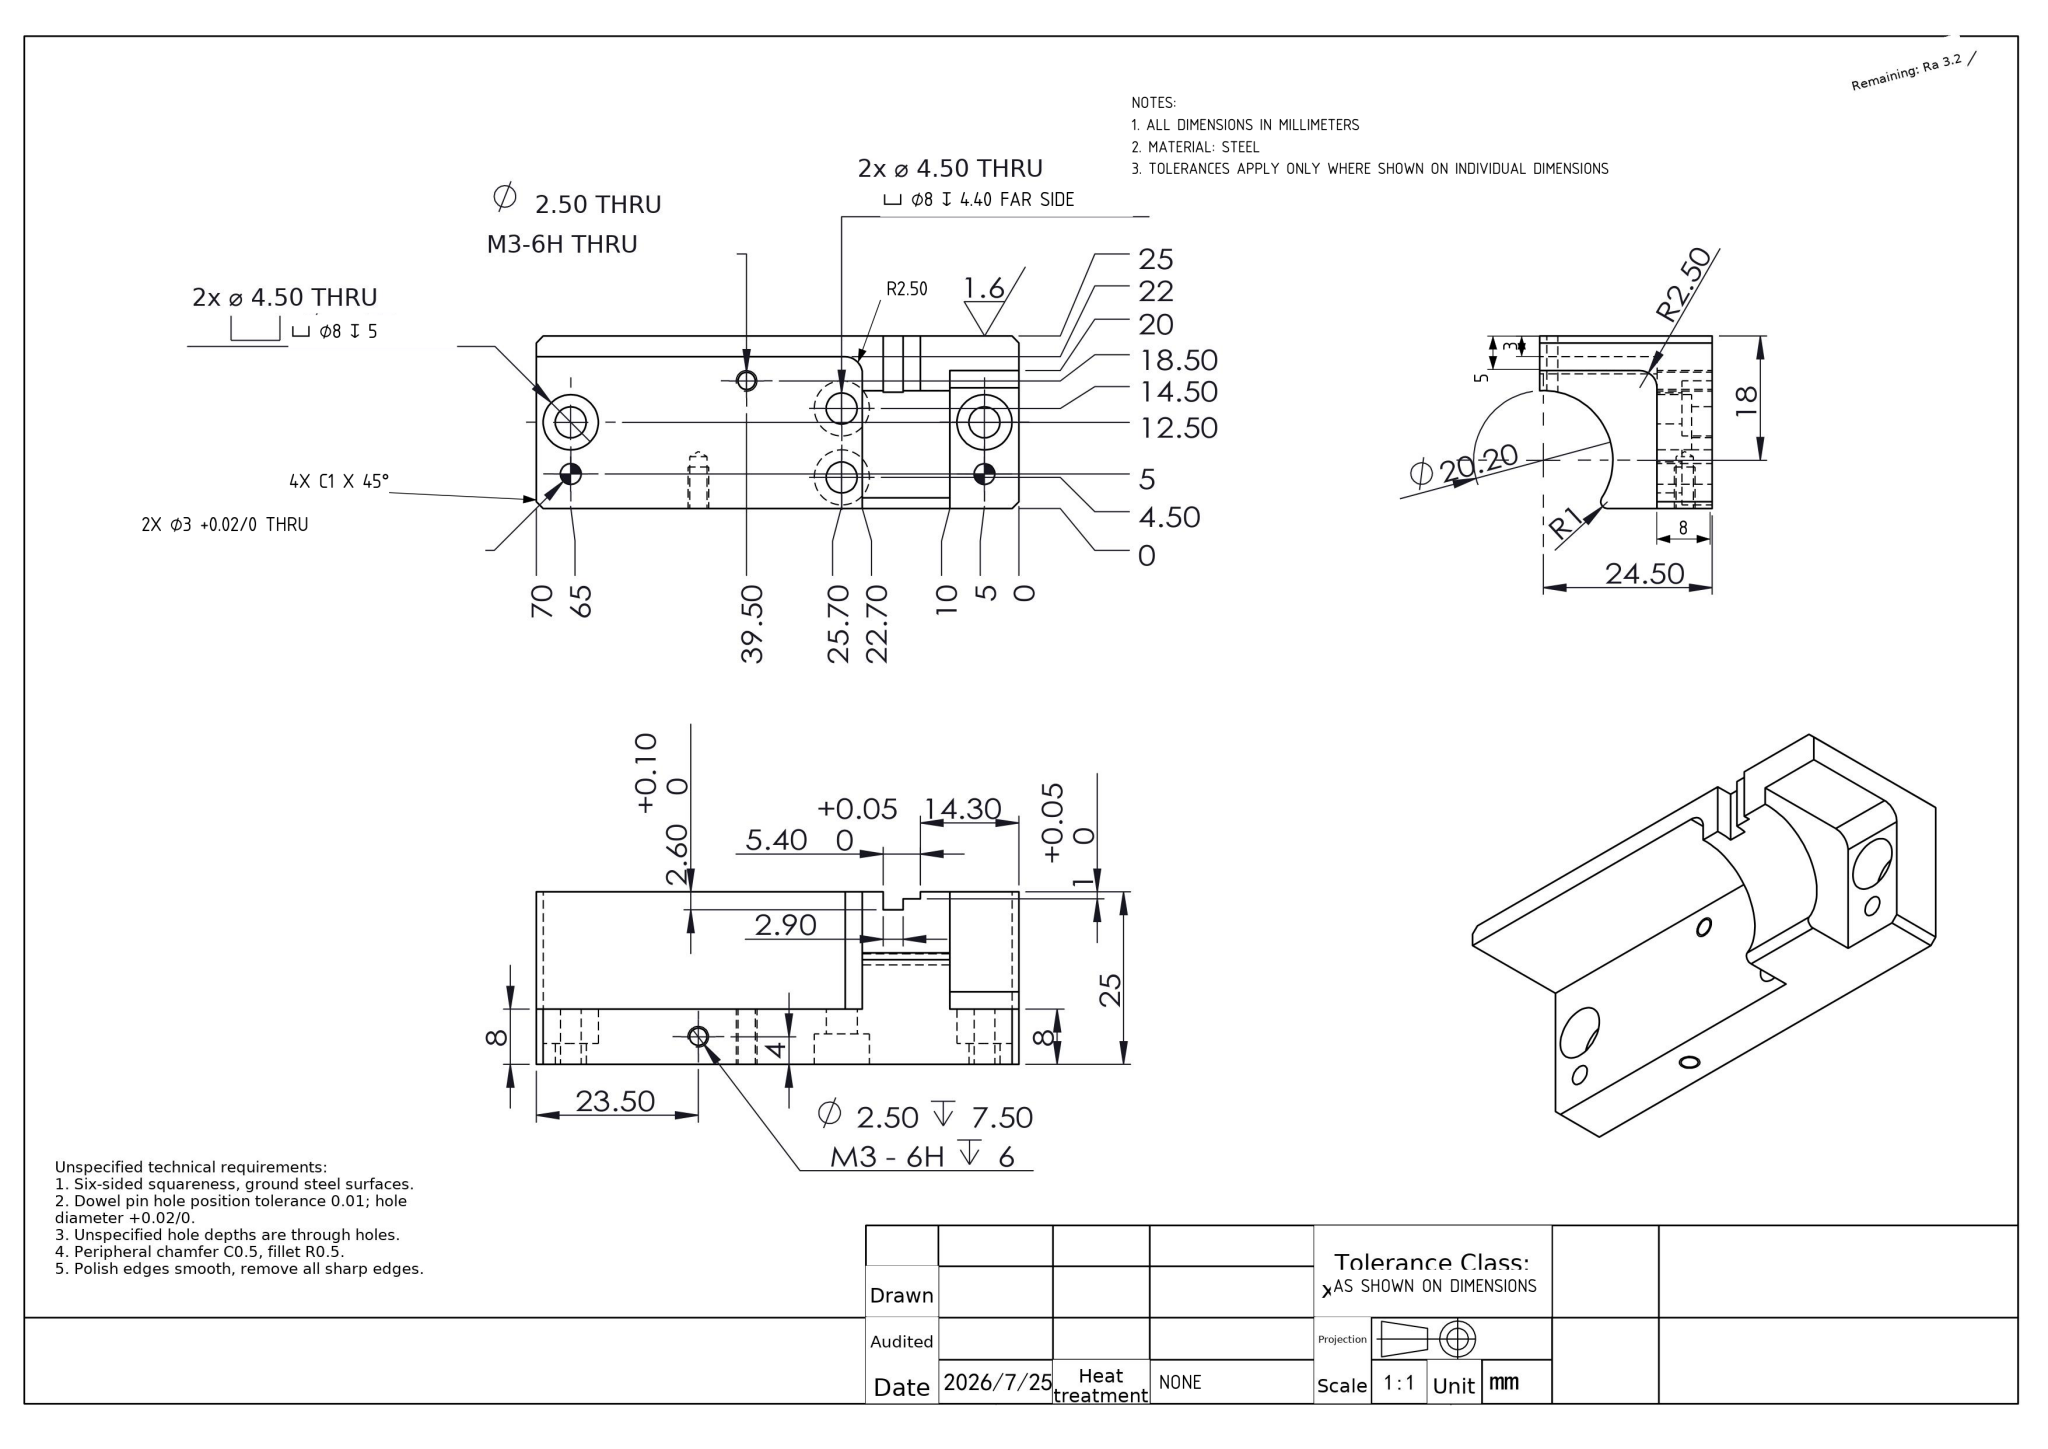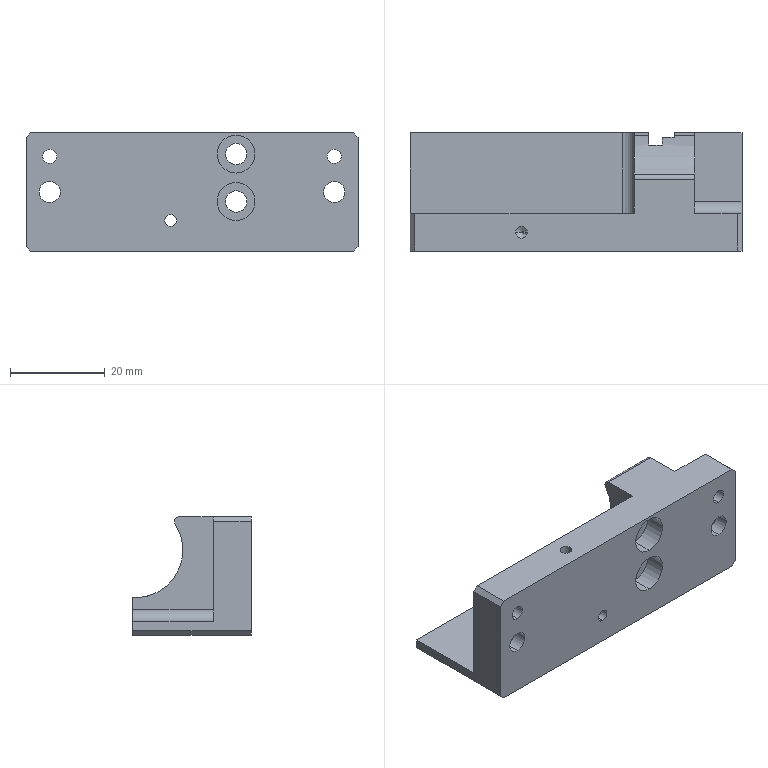Part | NX | mm | 1 solid | 58 faces | box 70 x 25 x 25 mm | volume 19281 mm3 | cylinder 30 | plane 26 | cone 2 | commonest cylinder face diameters 8 x8 4.5 x8 2.5 x4 3 x4 20.2 x3 5 x2 2 x1